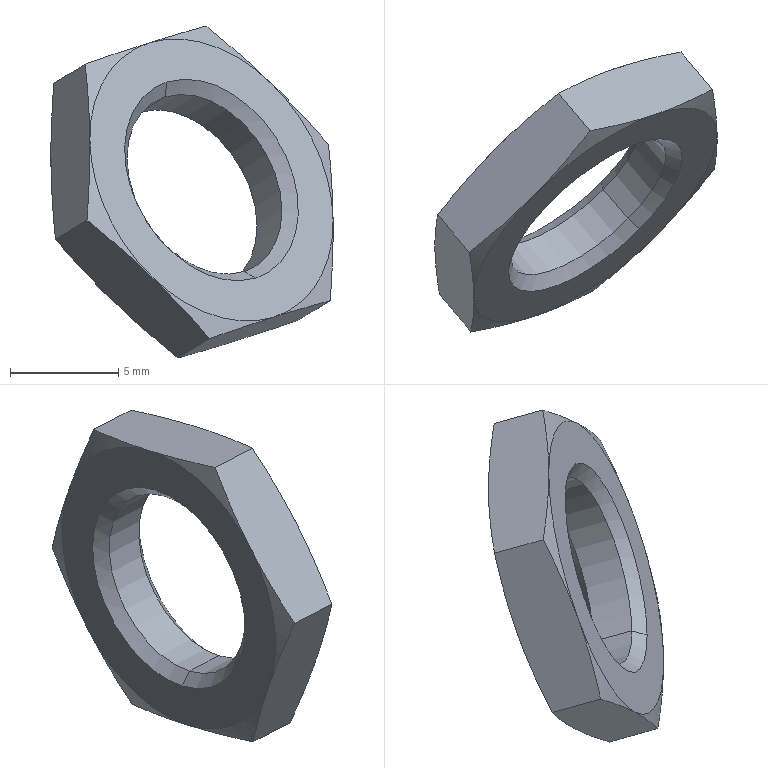Component | SolidWorks | SCPG-L-00-16-45-T0H-D-7_5-1 | 1 solid | 26 faces | box 13.01 x 12.91 x 15.3 mm | volume 310 mm3 | cone 16 | plane 8 | cylinder 2 | commonest cylinder face diameters 8.917 x2
STEP:
#1=COLOUR_RGB('',0.7922,0.8196,0.9333);
#2=FILL_AREA_STYLE_COLOUR('',#1);
#3=FILL_AREA_STYLE('',(#2));
#4=SURFACE_STYLE_FILL_AREA(#3);
#5=SURFACE_SIDE_STYLE('',(#4));
#6=SURFACE_STYLE_USAGE(.BOTH.,#5);
#7=PRESENTATION_STYLE_ASSIGNMENT((#6));
#8=CARTESIAN_POINT('',(17.404,-8.214,-2.973));
#9=VERTEX_POINT('',#8);
#10=CARTESIAN_POINT('',(17.548,-8.258,-3.29));
#11=VERTEX_POINT('',#10);
#12=CARTESIAN_POINT('',(17.476,-8.236,-3.132));
#13=DIRECTION('',(0.5985,-0.711,0.3692));
#14=DIRECTION('',(-0.6887,-0.692,-0.2163));
#15=AXIS2_PLACEMENT_3D('',#12,#13,#14);
#16=CIRCLE('',#15,0.1755);
#17=EDGE_CURVE('',#9,#11,#16,.T.);
#18=ORIENTED_EDGE('',*,*,#17,.F.);
#19=CARTESIAN_POINT('',(17.408,-8.226,-2.946));
#20=VERTEX_POINT('',#19);
#21=CARTESIAN_POINT('',(17.408,-8.226,-2.946));
#22=DIRECTION('',(0.1337,-0.4145,0.9002));
#23=VECTOR('',#22,39.37);
#24=LINE('',#21,#23);
#25=EDGE_CURVE('',#9,#20,#24,.T.);
#26=ORIENTED_EDGE('',*,*,#25,.T.);
#27=CARTESIAN_POINT('',(17.569,-8.275,-3.302));
#28=VERTEX_POINT('',#27);
#29=CARTESIAN_POINT('',(17.488,-8.251,-3.124));
#30=DIRECTION('',(-0.5985,0.711,-0.3692));
#31=DIRECTION('',(0.4093,-0.1248,-0.9038));
#32=AXIS2_PLACEMENT_3D('',#29,#30,#31);
#33=CIRCLE('',#32,0.1969);
#34=EDGE_CURVE('',#28,#20,#33,.T.);
#35=ORIENTED_EDGE('',*,*,#34,.F.);
#36=CARTESIAN_POINT('',(17.569,-8.275,-3.302));
#37=DIRECTION('',(0.7126,-0.591,-0.378));
#38=VECTOR('',#37,39.37);
#39=LINE('',#36,#38);
#40=EDGE_CURVE('',#11,#28,#39,.T.);
#41=ORIENTED_EDGE('',*,*,#40,.F.);
#42=EDGE_LOOP('',(#18,#26,#35,#41));
#43=FACE_OUTER_BOUND('',#42,.T.);
#44=CARTESIAN_POINT('',(17.488,-8.251,-3.124));
#45=DIRECTION('',(0.5985,-0.711,0.3692));
#46=DIRECTION('',(0.4093,-0.1248,-0.9038));
#47=AXIS2_PLACEMENT_3D('',#44,#45,#46);
#48=CONICAL_SURFACE('',#47,0.1969,0.7854);
#49=ADVANCED_FACE('',(#43),#48,.F.);
#50=ORIENTED_EDGE('',*,*,#17,.T.);
#51=CARTESIAN_POINT('',(17.502,-8.204,-3.318));
#52=VERTEX_POINT('',#51);
#53=CARTESIAN_POINT('',(17.525,-8.231,-3.304));
#54=DIRECTION('',(-0.5985,0.711,-0.3692));
#55=VECTOR('',#54,39.37);
#56=LINE('',#53,#55);
#57=EDGE_CURVE('',#11,#52,#56,.T.);
#58=ORIENTED_EDGE('',*,*,#57,.T.);
#59=CARTESIAN_POINT('',(17.359,-8.16,-3.001));
#60=VERTEX_POINT('',#59);
#61=CARTESIAN_POINT('',(17.43,-8.182,-3.159));
#62=DIRECTION('',(0.5985,-0.711,0.3692));
#63=DIRECTION('',(-0.4093,0.1248,0.9038));
#64=AXIS2_PLACEMENT_3D('',#61,#62,#63);
#65=CIRCLE('',#64,0.1755);
#66=EDGE_CURVE('',#60,#52,#65,.T.);
#67=ORIENTED_EDGE('',*,*,#66,.F.);
#68=CARTESIAN_POINT('',(17.381,-8.187,-2.987));
#69=DIRECTION('',(-0.5985,0.711,-0.3692));
#70=VECTOR('',#69,39.37);
#71=LINE('',#68,#70);
#72=EDGE_CURVE('',#9,#60,#71,.T.);
#73=ORIENTED_EDGE('',*,*,#72,.F.);
#74=EDGE_LOOP('',(#50,#58,#67,#73));
#75=FACE_OUTER_BOUND('',#74,.T.);
#76=CARTESIAN_POINT('',(17.453,-8.209,-3.146));
#77=DIRECTION('',(-0.5985,0.711,-0.3692));
#78=DIRECTION('',(-0.4093,0.1248,0.9038));
#79=AXIS2_PLACEMENT_3D('',#76,#77,#78);
#80=CYLINDRICAL_SURFACE('',#79,0.1755);
#81=ADVANCED_FACE('',(#75),#80,.F.);
#82=ORIENTED_EDGE('',*,*,#66,.T.);
#83=CARTESIAN_POINT('',(17.498,-8.191,-3.345));
#84=VERTEX_POINT('',#83);
#85=CARTESIAN_POINT('',(17.498,-8.191,-3.345));
#86=DIRECTION('',(-0.1337,0.4145,-0.9002));
#87=VECTOR('',#86,39.37);
#88=LINE('',#85,#87);
#89=EDGE_CURVE('',#52,#84,#88,.T.);
#90=ORIENTED_EDGE('',*,*,#89,.T.);
#91=CARTESIAN_POINT('',(17.337,-8.142,-2.989));
#92=VERTEX_POINT('',#91);
#93=CARTESIAN_POINT('',(17.418,-8.167,-3.167));
#94=DIRECTION('',(0.5985,-0.711,0.3692));
#95=DIRECTION('',(-0.4093,0.1248,0.9038));
#96=AXIS2_PLACEMENT_3D('',#93,#94,#95);
#97=CIRCLE('',#96,0.1969);
#98=EDGE_CURVE('',#92,#84,#97,.T.);
#99=ORIENTED_EDGE('',*,*,#98,.F.);
#100=CARTESIAN_POINT('',(17.337,-8.142,-2.989));
#101=DIRECTION('',(-0.7126,0.591,0.378));
#102=VECTOR('',#101,39.37);
#103=LINE('',#100,#102);
#104=EDGE_CURVE('',#60,#92,#103,.T.);
#105=ORIENTED_EDGE('',*,*,#104,.F.);
#106=EDGE_LOOP('',(#82,#90,#99,#105));
#107=FACE_OUTER_BOUND('',#106,.T.);
#108=CARTESIAN_POINT('',(17.418,-8.167,-3.167));
#109=DIRECTION('',(-0.5985,0.711,-0.3692));
#110=DIRECTION('',(-0.4093,0.1248,0.9038));
#111=AXIS2_PLACEMENT_3D('',#108,#109,#110);
#112=CONICAL_SURFACE('',#111,0.1969,0.7854);
#113=ADVANCED_FACE('',(#107),#112,.F.);
#114=CARTESIAN_POINT('',(17.596,-8.068,-2.948));
#115=VERTEX_POINT('',#114);
#116=CARTESIAN_POINT('',(17.376,-8.216,-2.875));
#117=VERTEX_POINT('',#116);
#118=CARTESIAN_POINT('',(17.488,-8.251,-3.124));
#119=DIRECTION('',(0.5985,-0.711,0.3692));
#120=DIRECTION('',(-0.4093,0.1248,0.9038));
#121=AXIS2_PLACEMENT_3D('',#118,#119,#120);
#122=CIRCLE('',#121,0.2756);
#123=EDGE_CURVE('',#115,#117,#122,.T.);
#124=ORIENTED_EDGE('',*,*,#123,.T.);
#125=CARTESIAN_POINT('',(17.268,-8.399,-3.051));
#126=VERTEX_POINT('',#125);
#127=CARTESIAN_POINT('',(17.488,-8.251,-3.124));
#128=DIRECTION('',(0.5985,-0.711,0.3692));
#129=DIRECTION('',(-0.4093,0.1248,0.9038));
#130=AXIS2_PLACEMENT_3D('',#127,#128,#129);
#131=CIRCLE('',#130,0.2756);
#132=EDGE_CURVE('',#117,#126,#131,.T.);
#133=ORIENTED_EDGE('',*,*,#132,.T.);
#134=CARTESIAN_POINT('',(17.38,-8.433,-3.3));
#135=VERTEX_POINT('',#134);
#136=CARTESIAN_POINT('',(17.488,-8.251,-3.124));
#137=DIRECTION('',(0.5985,-0.711,0.3692));
#138=DIRECTION('',(-0.4093,0.1248,0.9038));
#139=AXIS2_PLACEMENT_3D('',#136,#137,#138);
#140=CIRCLE('',#139,0.2756);
#141=EDGE_CURVE('',#126,#135,#140,.T.);
#142=ORIENTED_EDGE('',*,*,#141,.T.);
#143=CARTESIAN_POINT('',(17.601,-8.285,-3.373));
#144=VERTEX_POINT('',#143);
#145=CARTESIAN_POINT('',(17.488,-8.251,-3.124));
#146=DIRECTION('',(0.5985,-0.711,0.3692));
#147=DIRECTION('',(-0.4093,0.1248,0.9038));
#148=AXIS2_PLACEMENT_3D('',#145,#146,#147);
#149=CIRCLE('',#148,0.2756);
#150=EDGE_CURVE('',#135,#144,#149,.T.);
#151=ORIENTED_EDGE('',*,*,#150,.T.);
#152=CARTESIAN_POINT('',(17.709,-8.103,-3.197));
#153=VERTEX_POINT('',#152);
#154=CARTESIAN_POINT('',(17.488,-8.251,-3.124));
#155=DIRECTION('',(0.5985,-0.711,0.3692));
#156=DIRECTION('',(-0.4093,0.1248,0.9038));
#157=AXIS2_PLACEMENT_3D('',#154,#155,#156);
#158=CIRCLE('',#157,0.2756);
#159=EDGE_CURVE('',#144,#153,#158,.T.);
#160=ORIENTED_EDGE('',*,*,#159,.T.);
#161=CARTESIAN_POINT('',(17.488,-8.251,-3.124));
#162=DIRECTION('',(0.5985,-0.711,0.3692));
#163=DIRECTION('',(-0.4093,0.1248,0.9038));
#164=AXIS2_PLACEMENT_3D('',#161,#162,#163);
#165=CIRCLE('',#164,0.2756);
#166=EDGE_CURVE('',#153,#115,#165,.T.);
#167=ORIENTED_EDGE('',*,*,#166,.T.);
#168=EDGE_LOOP('',(#124,#133,#142,#151,#160,#167));
#169=FACE_OUTER_BOUND('',#168,.T.);
#170=ORIENTED_EDGE('',*,*,#34,.T.);
#171=CARTESIAN_POINT('',(17.488,-8.251,-3.124));
#172=DIRECTION('',(-0.5985,0.711,-0.3692));
#173=DIRECTION('',(0.4093,-0.1248,-0.9038));
#174=AXIS2_PLACEMENT_3D('',#171,#172,#173);
#175=CIRCLE('',#174,0.1969);
#176=EDGE_CURVE('',#20,#28,#175,.T.);
#177=ORIENTED_EDGE('',*,*,#176,.T.);
#178=EDGE_LOOP('',(#170,#177));
#179=FACE_BOUND('',#178,.T.);
#180=CARTESIAN_POINT('',(17.394,-8.346,-3.154));
#181=DIRECTION('',(0.5985,-0.711,0.3692));
#182=DIRECTION('',(0.4093,-0.1248,-0.9038));
#183=AXIS2_PLACEMENT_3D('',#180,#181,#182);
#184=PLANE('',#183);
#185=ADVANCED_FACE('',(#169,#179),#184,.T.);
#186=CARTESIAN_POINT('',(17.259,-8.318,-2.913));
#187=VERTEX_POINT('',#186);
#188=CARTESIAN_POINT('',(17.259,-8.318,-2.913));
#189=CARTESIAN_POINT('',(17.264,-8.347,-2.958));
#190=CARTESIAN_POINT('',(17.267,-8.375,-3.003));
#191=CARTESIAN_POINT('',(17.268,-8.399,-3.051));
#192=B_SPLINE_CURVE_WITH_KNOTS('',3,(#188,#189,#190,#191),.UNSPECIFIED.,.F.,.F.,(4,4),(0.,0.004052),.UNSPECIFIED.);
#193=EDGE_CURVE('',#187,#126,#192,.T.);
#194=ORIENTED_EDGE('',*,*,#193,.T.);
#195=ORIENTED_EDGE('',*,*,#132,.F.);
#196=CARTESIAN_POINT('',(17.376,-8.216,-2.875));
#197=CARTESIAN_POINT('',(17.339,-8.253,-2.886));
#198=CARTESIAN_POINT('',(17.3,-8.287,-2.899));
#199=CARTESIAN_POINT('',(17.259,-8.318,-2.913));
#200=B_SPLINE_CURVE_WITH_KNOTS('',3,(#196,#197,#198,#199),.UNSPECIFIED.,.F.,.F.,(4,4),(0.,0.004052),.UNSPECIFIED.);
#201=EDGE_CURVE('',#117,#187,#200,.T.);
#202=ORIENTED_EDGE('',*,*,#201,.T.);
#203=EDGE_LOOP('',(#194,#195,#202));
#204=FACE_OUTER_BOUND('',#203,.T.);
#205=CARTESIAN_POINT('',(17.482,-8.243,-3.128));
#206=DIRECTION('',(-0.5985,0.711,-0.3692));
#207=DIRECTION('',(-0.4093,0.1248,0.9038));
#208=AXIS2_PLACEMENT_3D('',#205,#206,#207);
#209=CONICAL_SURFACE('',#208,0.3185,1.309);
#210=ADVANCED_FACE('',(#204),#209,.T.);
#211=CARTESIAN_POINT('',(17.478,-8.098,-2.844));
#212=VERTEX_POINT('',#211);
#213=CARTESIAN_POINT('',(17.478,-8.098,-2.844));
#214=CARTESIAN_POINT('',(17.446,-8.14,-2.853));
#215=CARTESIAN_POINT('',(17.412,-8.179,-2.863));
#216=CARTESIAN_POINT('',(17.376,-8.216,-2.875));
#217=B_SPLINE_CURVE_WITH_KNOTS('',3,(#213,#214,#215,#216),.UNSPECIFIED.,.F.,.F.,(4,4),(0.,0.004052),.UNSPECIFIED.);
#218=EDGE_CURVE('',#212,#117,#217,.T.);
#219=ORIENTED_EDGE('',*,*,#218,.T.);
#220=ORIENTED_EDGE('',*,*,#123,.F.);
#221=CARTESIAN_POINT('',(17.596,-8.068,-2.948));
#222=CARTESIAN_POINT('',(17.559,-8.081,-2.912));
#223=CARTESIAN_POINT('',(17.519,-8.091,-2.877));
#224=CARTESIAN_POINT('',(17.478,-8.098,-2.844));
#225=B_SPLINE_CURVE_WITH_KNOTS('',3,(#221,#222,#223,#224),.UNSPECIFIED.,.F.,.F.,(4,4),(0.,0.004052),.UNSPECIFIED.);
#226=EDGE_CURVE('',#115,#212,#225,.T.);
#227=ORIENTED_EDGE('',*,*,#226,.T.);
#228=EDGE_LOOP('',(#219,#220,#227));
#229=FACE_OUTER_BOUND('',#228,.T.);
#230=CARTESIAN_POINT('',(17.482,-8.243,-3.128));
#231=DIRECTION('',(-0.5985,0.711,-0.3692));
#232=DIRECTION('',(-0.4093,0.1248,0.9038));
#233=AXIS2_PLACEMENT_3D('',#230,#231,#232);
#234=CONICAL_SURFACE('',#233,0.3185,1.309);
#235=ADVANCED_FACE('',(#229),#234,.T.);
#236=CARTESIAN_POINT('',(17.701,-8.022,-3.059));
#237=VERTEX_POINT('',#236);
#238=CARTESIAN_POINT('',(17.701,-8.022,-3.059));
#239=CARTESIAN_POINT('',(17.668,-8.04,-3.021));
#240=CARTESIAN_POINT('',(17.634,-8.056,-2.983));
#241=CARTESIAN_POINT('',(17.596,-8.068,-2.948));
#242=B_SPLINE_CURVE_WITH_KNOTS('',3,(#238,#239,#240,#241),.UNSPECIFIED.,.F.,.F.,(4,4),(0.,0.004052),.UNSPECIFIED.);
#243=EDGE_CURVE('',#237,#115,#242,.T.);
#244=ORIENTED_EDGE('',*,*,#243,.T.);
#245=ORIENTED_EDGE('',*,*,#166,.F.);
#246=CARTESIAN_POINT('',(17.709,-8.103,-3.197));
#247=CARTESIAN_POINT('',(17.709,-8.079,-3.149));
#248=CARTESIAN_POINT('',(17.706,-8.051,-3.104));
#249=CARTESIAN_POINT('',(17.701,-8.022,-3.059));
#250=B_SPLINE_CURVE_WITH_KNOTS('',3,(#246,#247,#248,#249),.UNSPECIFIED.,.F.,.F.,(4,4),(0.,0.004052),.UNSPECIFIED.);
#251=EDGE_CURVE('',#153,#237,#250,.T.);
#252=ORIENTED_EDGE('',*,*,#251,.T.);
#253=EDGE_LOOP('',(#244,#245,#252));
#254=FACE_OUTER_BOUND('',#253,.T.);
#255=CARTESIAN_POINT('',(17.482,-8.243,-3.128));
#256=DIRECTION('',(-0.5985,0.711,-0.3692));
#257=DIRECTION('',(-0.4093,0.1248,0.9038));
#258=AXIS2_PLACEMENT_3D('',#255,#256,#257);
#259=CONICAL_SURFACE('',#258,0.3185,1.309);
#260=ADVANCED_FACE('',(#254),#259,.T.);
#261=ORIENTED_EDGE('',*,*,#159,.F.);
#262=CARTESIAN_POINT('',(17.704,-8.167,-3.343));
#263=VERTEX_POINT('',#262);
#264=CARTESIAN_POINT('',(17.601,-8.285,-3.373));
#265=CARTESIAN_POINT('',(17.638,-8.248,-3.361));
#266=CARTESIAN_POINT('',(17.672,-8.209,-3.351));
#267=CARTESIAN_POINT('',(17.704,-8.167,-3.343));
#268=B_SPLINE_CURVE_WITH_KNOTS('',3,(#264,#265,#266,#267),.UNSPECIFIED.,.F.,.F.,(4,4),(0.,0.004052),.UNSPECIFIED.);
#269=EDGE_CURVE('',#144,#263,#268,.T.);
#270=ORIENTED_EDGE('',*,*,#269,.T.);
#271=CARTESIAN_POINT('',(17.704,-8.167,-3.343));
#272=CARTESIAN_POINT('',(17.708,-8.148,-3.293));
#273=CARTESIAN_POINT('',(17.71,-8.127,-3.244));
#274=CARTESIAN_POINT('',(17.709,-8.103,-3.197));
#275=B_SPLINE_CURVE_WITH_KNOTS('',3,(#271,#272,#273,#274),.UNSPECIFIED.,.F.,.F.,(4,4),(0.,0.004052),.UNSPECIFIED.);
#276=EDGE_CURVE('',#263,#153,#275,.T.);
#277=ORIENTED_EDGE('',*,*,#276,.T.);
#278=EDGE_LOOP('',(#261,#270,#277));
#279=FACE_OUTER_BOUND('',#278,.T.);
#280=CARTESIAN_POINT('',(17.482,-8.243,-3.128));
#281=DIRECTION('',(-0.5985,0.711,-0.3692));
#282=DIRECTION('',(-0.4093,0.1248,0.9038));
#283=AXIS2_PLACEMENT_3D('',#280,#281,#282);
#284=CONICAL_SURFACE('',#283,0.3185,1.309);
#285=ADVANCED_FACE('',(#279),#284,.T.);
#286=ORIENTED_EDGE('',*,*,#150,.F.);
#287=CARTESIAN_POINT('',(17.485,-8.387,-3.411));
#288=VERTEX_POINT('',#287);
#289=CARTESIAN_POINT('',(17.38,-8.433,-3.3));
#290=CARTESIAN_POINT('',(17.418,-8.42,-3.336));
#291=CARTESIAN_POINT('',(17.452,-8.405,-3.373));
#292=CARTESIAN_POINT('',(17.485,-8.387,-3.411));
#293=B_SPLINE_CURVE_WITH_KNOTS('',3,(#289,#290,#291,#292),.UNSPECIFIED.,.F.,.F.,(4,4),(0.,0.004052),.UNSPECIFIED.);
#294=EDGE_CURVE('',#135,#288,#293,.T.);
#295=ORIENTED_EDGE('',*,*,#294,.T.);
#296=CARTESIAN_POINT('',(17.485,-8.387,-3.411));
#297=CARTESIAN_POINT('',(17.525,-8.356,-3.397));
#298=CARTESIAN_POINT('',(17.565,-8.322,-3.384));
#299=CARTESIAN_POINT('',(17.601,-8.285,-3.373));
#300=B_SPLINE_CURVE_WITH_KNOTS('',3,(#296,#297,#298,#299),.UNSPECIFIED.,.F.,.F.,(4,4),(0.,0.004052),.UNSPECIFIED.);
#301=EDGE_CURVE('',#288,#144,#300,.T.);
#302=ORIENTED_EDGE('',*,*,#301,.T.);
#303=EDGE_LOOP('',(#286,#295,#302));
#304=FACE_OUTER_BOUND('',#303,.T.);
#305=CARTESIAN_POINT('',(17.482,-8.243,-3.128));
#306=DIRECTION('',(-0.5985,0.711,-0.3692));
#307=DIRECTION('',(-0.4093,0.1248,0.9038));
#308=AXIS2_PLACEMENT_3D('',#305,#306,#307);
#309=CONICAL_SURFACE('',#308,0.3185,1.309);
#310=ADVANCED_FACE('',(#304),#309,.T.);
#311=CARTESIAN_POINT('',(17.262,-8.463,-3.197));
#312=VERTEX_POINT('',#311);
#313=CARTESIAN_POINT('',(17.262,-8.463,-3.197));
#314=CARTESIAN_POINT('',(17.304,-8.455,-3.23));
#315=CARTESIAN_POINT('',(17.343,-8.446,-3.264));
#316=CARTESIAN_POINT('',(17.38,-8.433,-3.3));
#317=B_SPLINE_CURVE_WITH_KNOTS('',3,(#313,#314,#315,#316),.UNSPECIFIED.,.F.,.F.,(4,4),(0.,0.004052),.UNSPECIFIED.);
#318=EDGE_CURVE('',#312,#135,#317,.T.);
#319=ORIENTED_EDGE('',*,*,#318,.T.);
#320=ORIENTED_EDGE('',*,*,#141,.F.);
#321=CARTESIAN_POINT('',(17.268,-8.399,-3.051));
#322=CARTESIAN_POINT('',(17.268,-8.423,-3.098));
#323=CARTESIAN_POINT('',(17.266,-8.444,-3.147));
#324=CARTESIAN_POINT('',(17.262,-8.463,-3.197));
#325=B_SPLINE_CURVE_WITH_KNOTS('',3,(#321,#322,#323,#324),.UNSPECIFIED.,.F.,.F.,(4,4),(0.,0.004052),.UNSPECIFIED.);
#326=EDGE_CURVE('',#126,#312,#325,.T.);
#327=ORIENTED_EDGE('',*,*,#326,.T.);
#328=EDGE_LOOP('',(#319,#320,#327));
#329=FACE_OUTER_BOUND('',#328,.T.);
#330=CARTESIAN_POINT('',(17.482,-8.243,-3.128));
#331=DIRECTION('',(-0.5985,0.711,-0.3692));
#332=DIRECTION('',(-0.4093,0.1248,0.9038));
#333=AXIS2_PLACEMENT_3D('',#330,#331,#332);
#334=CONICAL_SURFACE('',#333,0.3185,1.309);
#335=ADVANCED_FACE('',(#329),#334,.T.);
#336=ORIENTED_EDGE('',*,*,#25,.F.);
#337=CARTESIAN_POINT('',(17.476,-8.236,-3.132));
#338=DIRECTION('',(0.5985,-0.711,0.3692));
#339=DIRECTION('',(-0.6887,-0.692,-0.2163));
#340=AXIS2_PLACEMENT_3D('',#337,#338,#339);
#341=CIRCLE('',#340,0.1755);
#342=EDGE_CURVE('',#11,#9,#341,.T.);
#343=ORIENTED_EDGE('',*,*,#342,.F.);
#344=ORIENTED_EDGE('',*,*,#40,.T.);
#345=ORIENTED_EDGE('',*,*,#176,.F.);
#346=EDGE_LOOP('',(#336,#343,#344,#345));
#347=FACE_OUTER_BOUND('',#346,.T.);
#348=CARTESIAN_POINT('',(17.488,-8.251,-3.124));
#349=DIRECTION('',(0.5985,-0.711,0.3692));
#350=DIRECTION('',(0.4093,-0.1248,-0.9038));
#351=AXIS2_PLACEMENT_3D('',#348,#349,#350);
#352=CONICAL_SURFACE('',#351,0.1969,0.7854);
#353=ADVANCED_FACE('',(#347),#352,.F.);
#354=CARTESIAN_POINT('',(17.205,-8.395,-3.232));
#355=VERTEX_POINT('',#354);
#356=CARTESIAN_POINT('',(17.269,-8.471,-3.193));
#357=DIRECTION('',(-0.5985,0.711,-0.3692));
#358=VECTOR('',#357,39.37);
#359=LINE('',#356,#358);
#360=EDGE_CURVE('',#312,#355,#359,.T.);
#361=ORIENTED_EDGE('',*,*,#360,.F.);
#362=ORIENTED_EDGE('',*,*,#326,.F.);
#363=ORIENTED_EDGE('',*,*,#193,.F.);
#364=CARTESIAN_POINT('',(17.202,-8.251,-2.948));
#365=VERTEX_POINT('',#364);
#366=CARTESIAN_POINT('',(17.266,-8.326,-2.909));
#367=DIRECTION('',(0.5985,-0.711,0.3692));
#368=VECTOR('',#367,39.37);
#369=LINE('',#366,#368);
#370=EDGE_CURVE('',#365,#187,#369,.T.);
#371=ORIENTED_EDGE('',*,*,#370,.F.);
#372=CARTESIAN_POINT('',(17.197,-8.315,-3.094));
#373=VERTEX_POINT('',#372);
#374=CARTESIAN_POINT('',(17.197,-8.315,-3.094));
#375=CARTESIAN_POINT('',(17.196,-8.291,-3.047));
#376=CARTESIAN_POINT('',(17.198,-8.27,-2.998));
#377=CARTESIAN_POINT('',(17.202,-8.251,-2.948));
#378=B_SPLINE_CURVE_WITH_KNOTS('',3,(#374,#375,#376,#377),.UNSPECIFIED.,.F.,.F.,(4,4),(0.,0.004052),.UNSPECIFIED.);
#379=EDGE_CURVE('',#373,#365,#378,.T.);
#380=ORIENTED_EDGE('',*,*,#379,.F.);
#381=CARTESIAN_POINT('',(17.205,-8.395,-3.232));
#382=CARTESIAN_POINT('',(17.201,-8.366,-3.188));
#383=CARTESIAN_POINT('',(17.198,-8.339,-3.142));
#384=CARTESIAN_POINT('',(17.197,-8.315,-3.094));
#385=B_SPLINE_CURVE_WITH_KNOTS('',3,(#381,#382,#383,#384),.UNSPECIFIED.,.F.,.F.,(4,4),(0.,0.004052),.UNSPECIFIED.);
#386=EDGE_CURVE('',#355,#373,#385,.T.);
#387=ORIENTED_EDGE('',*,*,#386,.F.);
#388=EDGE_LOOP('',(#361,#362,#363,#371,#380,#387));
#389=FACE_OUTER_BOUND('',#388,.T.);
#390=CARTESIAN_POINT('',(17.269,-8.471,-3.193));
#391=DIRECTION('',(0.8011,0.5369,-0.2645));
#392=DIRECTION('',(0.01014,-0.4541,-0.8909));
#393=AXIS2_PLACEMENT_3D('',#390,#391,#392);
#394=PLANE('',#393);
#395=ADVANCED_FACE('',(#389),#394,.F.);
#396=CARTESIAN_POINT('',(17.305,-8.132,-2.918));
#397=VERTEX_POINT('',#396);
#398=CARTESIAN_POINT('',(17.202,-8.251,-2.948));
#399=CARTESIAN_POINT('',(17.234,-8.209,-2.94));
#400=CARTESIAN_POINT('',(17.268,-8.169,-2.93));
#401=CARTESIAN_POINT('',(17.305,-8.132,-2.918));
#402=B_SPLINE_CURVE_WITH_KNOTS('',3,(#398,#399,#400,#401),.UNSPECIFIED.,.F.,.F.,(4,4),(0.,0.004052),.UNSPECIFIED.);
#403=EDGE_CURVE('',#365,#397,#402,.T.);
#404=ORIENTED_EDGE('',*,*,#403,.F.);
#405=ORIENTED_EDGE('',*,*,#370,.T.);
#406=ORIENTED_EDGE('',*,*,#201,.F.);
#407=ORIENTED_EDGE('',*,*,#218,.F.);
#408=CARTESIAN_POINT('',(17.421,-8.03,-2.88));
#409=VERTEX_POINT('',#408);
#410=CARTESIAN_POINT('',(17.485,-8.106,-2.84));
#411=DIRECTION('',(0.5985,-0.711,0.3692));
#412=VECTOR('',#411,39.37);
#413=LINE('',#410,#412);
#414=EDGE_CURVE('',#409,#212,#413,.T.);
#415=ORIENTED_EDGE('',*,*,#414,.F.);
#416=CARTESIAN_POINT('',(17.305,-8.132,-2.918));
#417=CARTESIAN_POINT('',(17.342,-8.096,-2.907));
#418=CARTESIAN_POINT('',(17.381,-8.062,-2.894));
#419=CARTESIAN_POINT('',(17.421,-8.03,-2.88));
#420=B_SPLINE_CURVE_WITH_KNOTS('',3,(#416,#417,#418,#419),.UNSPECIFIED.,.F.,.F.,(4,4),(0.,0.004052),.UNSPECIFIED.);
#421=EDGE_CURVE('',#397,#409,#420,.T.);
#422=ORIENTED_EDGE('',*,*,#421,.F.);
#423=EDGE_LOOP('',(#404,#405,#406,#407,#415,#422));
#424=FACE_OUTER_BOUND('',#423,.T.);
#425=CARTESIAN_POINT('',(17.266,-8.326,-2.909));
#426=DIRECTION('',(0.4093,-0.1248,-0.9038));
#427=DIRECTION('',(-0.5985,0.711,-0.3692));
#428=AXIS2_PLACEMENT_3D('',#425,#426,#427);
#429=PLANE('',#428);
#430=ADVANCED_FACE('',(#424),#429,.F.);
#431=CARTESIAN_POINT('',(17.526,-7.984,-2.991));
#432=VERTEX_POINT('',#431);
#433=CARTESIAN_POINT('',(17.421,-8.03,-2.88));
#434=CARTESIAN_POINT('',(17.454,-8.013,-2.918));
#435=CARTESIAN_POINT('',(17.488,-7.997,-2.955));
#436=CARTESIAN_POINT('',(17.526,-7.984,-2.991));
#437=B_SPLINE_CURVE_WITH_KNOTS('',3,(#433,#434,#435,#436),.UNSPECIFIED.,.F.,.F.,(4,4),(0.,0.004052),.UNSPECIFIED.);
#438=EDGE_CURVE('',#409,#432,#437,.T.);
#439=ORIENTED_EDGE('',*,*,#438,.F.);
#440=ORIENTED_EDGE('',*,*,#414,.T.);
#441=ORIENTED_EDGE('',*,*,#226,.F.);
#442=ORIENTED_EDGE('',*,*,#243,.F.);
#443=CARTESIAN_POINT('',(17.644,-7.955,-3.094));
#444=VERTEX_POINT('',#443);
#445=CARTESIAN_POINT('',(17.708,-8.031,-3.055));
#446=DIRECTION('',(0.5985,-0.711,0.3692));
#447=VECTOR('',#446,39.37);
#448=LINE('',#445,#447);
#449=EDGE_CURVE('',#444,#237,#448,.T.);
#450=ORIENTED_EDGE('',*,*,#449,.F.);
#451=CARTESIAN_POINT('',(17.526,-7.984,-2.991));
#452=CARTESIAN_POINT('',(17.563,-7.972,-3.027));
#453=CARTESIAN_POINT('',(17.603,-7.962,-3.061));
#454=CARTESIAN_POINT('',(17.644,-7.955,-3.094));
#455=B_SPLINE_CURVE_WITH_KNOTS('',3,(#451,#452,#453,#454),.UNSPECIFIED.,.F.,.F.,(4,4),(0.,0.004052),.UNSPECIFIED.);
#456=EDGE_CURVE('',#432,#444,#455,.T.);
#457=ORIENTED_EDGE('',*,*,#456,.F.);
#458=EDGE_LOOP('',(#439,#440,#441,#442,#450,#457));
#459=FACE_OUTER_BOUND('',#458,.T.);
#460=CARTESIAN_POINT('',(17.485,-8.106,-2.84));
#461=DIRECTION('',(-0.3918,-0.6617,-0.6393));
#462=DIRECTION('',(-0.6988,-0.2379,0.6745));
#463=AXIS2_PLACEMENT_3D('',#460,#461,#462);
#464=PLANE('',#463);
#465=ADVANCED_FACE('',(#459),#464,.F.);
#466=CARTESIAN_POINT('',(17.639,-8.019,-3.24));
#467=VERTEX_POINT('',#466);
#468=CARTESIAN_POINT('',(17.644,-7.955,-3.094));
#469=CARTESIAN_POINT('',(17.64,-7.974,-3.144));
#470=CARTESIAN_POINT('',(17.638,-7.995,-3.193));
#471=CARTESIAN_POINT('',(17.639,-8.019,-3.24));
#472=B_SPLINE_CURVE_WITH_KNOTS('',3,(#468,#469,#470,#471),.UNSPECIFIED.,.F.,.F.,(4,4),(0.,0.004052),.UNSPECIFIED.);
#473=EDGE_CURVE('',#444,#467,#472,.T.);
#474=ORIENTED_EDGE('',*,*,#473,.F.);
#475=ORIENTED_EDGE('',*,*,#449,.T.);
#476=ORIENTED_EDGE('',*,*,#251,.F.);
#477=ORIENTED_EDGE('',*,*,#276,.F.);
#478=CARTESIAN_POINT('',(17.647,-8.099,-3.378));
#479=VERTEX_POINT('',#478);
#480=CARTESIAN_POINT('',(17.711,-8.175,-3.338));
#481=DIRECTION('',(0.5985,-0.711,0.3692));
#482=VECTOR('',#481,39.37);
#483=LINE('',#480,#482);
#484=EDGE_CURVE('',#479,#263,#483,.T.);
#485=ORIENTED_EDGE('',*,*,#484,.F.);
#486=CARTESIAN_POINT('',(17.639,-8.019,-3.24));
#487=CARTESIAN_POINT('',(17.639,-8.043,-3.288));
#488=CARTESIAN_POINT('',(17.642,-8.07,-3.333));
#489=CARTESIAN_POINT('',(17.647,-8.099,-3.378));
#490=B_SPLINE_CURVE_WITH_KNOTS('',3,(#486,#487,#488,#489),.UNSPECIFIED.,.F.,.F.,(4,4),(0.,0.004052),.UNSPECIFIED.);
#491=EDGE_CURVE('',#467,#479,#490,.T.);
#492=ORIENTED_EDGE('',*,*,#491,.F.);
#493=EDGE_LOOP('',(#474,#475,#476,#477,#485,#492));
#494=FACE_OUTER_BOUND('',#493,.T.);
#495=CARTESIAN_POINT('',(17.708,-8.031,-3.055));
#496=DIRECTION('',(-0.8011,-0.5369,0.2645));
#497=DIRECTION('',(-0.01014,0.4541,0.8909));
#498=AXIS2_PLACEMENT_3D('',#495,#496,#497);
#499=PLANE('',#498);
#500=ADVANCED_FACE('',(#494),#499,.F.);
#501=ORIENTED_EDGE('',*,*,#484,.T.);
#502=ORIENTED_EDGE('',*,*,#269,.F.);
#503=ORIENTED_EDGE('',*,*,#301,.F.);
#504=CARTESIAN_POINT('',(17.428,-8.319,-3.447));
#505=VERTEX_POINT('',#504);
#506=CARTESIAN_POINT('',(17.492,-8.395,-3.407));
#507=DIRECTION('',(0.5985,-0.711,0.3692));
#508=VECTOR('',#507,39.37);
#509=LINE('',#506,#508);
#510=EDGE_CURVE('',#505,#288,#509,.T.);
#511=ORIENTED_EDGE('',*,*,#510,.F.);
#512=CARTESIAN_POINT('',(17.531,-8.201,-3.416));
#513=VERTEX_POINT('',#512);
#514=CARTESIAN_POINT('',(17.531,-8.201,-3.416));
#515=CARTESIAN_POINT('',(17.494,-8.238,-3.428));
#516=CARTESIAN_POINT('',(17.46,-8.278,-3.438));
#517=CARTESIAN_POINT('',(17.428,-8.319,-3.447));
#518=B_SPLINE_CURVE_WITH_KNOTS('',3,(#514,#515,#516,#517),.UNSPECIFIED.,.F.,.F.,(4,4),(0.,0.004052),.UNSPECIFIED.);
#519=EDGE_CURVE('',#513,#505,#518,.T.);
#520=ORIENTED_EDGE('',*,*,#519,.F.);
#521=CARTESIAN_POINT('',(17.647,-8.099,-3.378));
#522=CARTESIAN_POINT('',(17.606,-8.131,-3.392));
#523=CARTESIAN_POINT('',(17.567,-8.164,-3.405));
#524=CARTESIAN_POINT('',(17.531,-8.201,-3.416));
#525=B_SPLINE_CURVE_WITH_KNOTS('',3,(#521,#522,#523,#524),.UNSPECIFIED.,.F.,.F.,(4,4),(0.,0.004052),.UNSPECIFIED.);
#526=EDGE_CURVE('',#479,#513,#525,.T.);
#527=ORIENTED_EDGE('',*,*,#526,.F.);
#528=EDGE_LOOP('',(#501,#502,#503,#511,#520,#527));
#529=FACE_OUTER_BOUND('',#528,.T.);
#530=CARTESIAN_POINT('',(17.711,-8.175,-3.338));
#531=DIRECTION('',(-0.4093,0.1248,0.9038));
#532=DIRECTION('',(0.5985,-0.711,0.3692));
#533=AXIS2_PLACEMENT_3D('',#530,#531,#532);
#534=PLANE('',#533);
#535=ADVANCED_FACE('',(#529),#534,.F.);
#536=ORIENTED_EDGE('',*,*,#510,.T.);
#537=ORIENTED_EDGE('',*,*,#294,.F.);
#538=ORIENTED_EDGE('',*,*,#318,.F.);
#539=ORIENTED_EDGE('',*,*,#360,.T.);
#540=CARTESIAN_POINT('',(17.31,-8.349,-3.343));
#541=VERTEX_POINT('',#540);
#542=CARTESIAN_POINT('',(17.31,-8.349,-3.343));
#543=CARTESIAN_POINT('',(17.273,-8.362,-3.308));
#544=CARTESIAN_POINT('',(17.238,-8.378,-3.27));
#545=CARTESIAN_POINT('',(17.205,-8.395,-3.232));
#546=B_SPLINE_CURVE_WITH_KNOTS('',3,(#542,#543,#544,#545),.UNSPECIFIED.,.F.,.F.,(4,4),(0.,0.004052),.UNSPECIFIED.);
#547=EDGE_CURVE('',#541,#355,#546,.T.);
#548=ORIENTED_EDGE('',*,*,#547,.F.);
#549=CARTESIAN_POINT('',(17.428,-8.319,-3.447));
#550=CARTESIAN_POINT('',(17.387,-8.327,-3.414));
#551=CARTESIAN_POINT('',(17.347,-8.336,-3.379));
#552=CARTESIAN_POINT('',(17.31,-8.349,-3.343));
#553=B_SPLINE_CURVE_WITH_KNOTS('',3,(#549,#550,#551,#552),.UNSPECIFIED.,.F.,.F.,(4,4),(0.,0.004052),.UNSPECIFIED.);
#554=EDGE_CURVE('',#505,#541,#553,.T.);
#555=ORIENTED_EDGE('',*,*,#554,.F.);
#556=EDGE_LOOP('',(#536,#537,#538,#539,#548,#555));
#557=FACE_OUTER_BOUND('',#556,.T.);
#558=CARTESIAN_POINT('',(17.492,-8.395,-3.407));
#559=DIRECTION('',(0.3918,0.6617,0.6393));
#560=DIRECTION('',(0.6988,0.2379,-0.6745));
#561=AXIS2_PLACEMENT_3D('',#558,#559,#560);
#562=PLANE('',#561);
#563=ADVANCED_FACE('',(#557),#562,.F.);
#564=ORIENTED_EDGE('',*,*,#57,.F.);
#565=ORIENTED_EDGE('',*,*,#342,.T.);
#566=ORIENTED_EDGE('',*,*,#72,.T.);
#567=CARTESIAN_POINT('',(17.43,-8.182,-3.159));
#568=DIRECTION('',(0.5985,-0.711,0.3692));
#569=DIRECTION('',(-0.4093,0.1248,0.9038));
#570=AXIS2_PLACEMENT_3D('',#567,#568,#569);
#571=CIRCLE('',#570,0.1755);
#572=EDGE_CURVE('',#52,#60,#571,.T.);
#573=ORIENTED_EDGE('',*,*,#572,.F.);
#574=EDGE_LOOP('',(#564,#565,#566,#573));
#575=FACE_OUTER_BOUND('',#574,.T.);
#576=CARTESIAN_POINT('',(17.453,-8.209,-3.146));
#577=DIRECTION('',(-0.5985,0.711,-0.3692));
#578=DIRECTION('',(-0.4093,0.1248,0.9038));
#579=AXIS2_PLACEMENT_3D('',#576,#577,#578);
#580=CYLINDRICAL_SURFACE('',#579,0.1755);
#581=ADVANCED_FACE('',(#575),#580,.F.);
#582=ORIENTED_EDGE('',*,*,#386,.T.);
#583=CARTESIAN_POINT('',(17.418,-8.167,-3.167));
#584=DIRECTION('',(0.5985,-0.711,0.3692));
#585=DIRECTION('',(0.4093,-0.1248,-0.9038));
#586=AXIS2_PLACEMENT_3D('',#583,#584,#585);
#587=CIRCLE('',#586,0.2756);
#588=EDGE_CURVE('',#373,#541,#587,.T.);
#589=ORIENTED_EDGE('',*,*,#588,.T.);
#590=ORIENTED_EDGE('',*,*,#547,.T.);
#591=EDGE_LOOP('',(#582,#589,#590));
#592=FACE_OUTER_BOUND('',#591,.T.);
#593=CARTESIAN_POINT('',(17.425,-8.175,-3.163));
#594=DIRECTION('',(0.5985,-0.711,0.3692));
#595=DIRECTION('',(0.4093,-0.1248,-0.9038));
#596=AXIS2_PLACEMENT_3D('',#593,#594,#595);
#597=CONICAL_SURFACE('',#596,0.3185,1.309);
#598=ADVANCED_FACE('',(#592),#597,.T.);
#599=ORIENTED_EDGE('',*,*,#403,.T.);
#600=CARTESIAN_POINT('',(17.418,-8.167,-3.167));
#601=DIRECTION('',(0.5985,-0.711,0.3692));
#602=DIRECTION('',(0.4093,-0.1248,-0.9038));
#603=AXIS2_PLACEMENT_3D('',#600,#601,#602);
#604=CIRCLE('',#603,0.2756);
#605=EDGE_CURVE('',#397,#373,#604,.T.);
#606=ORIENTED_EDGE('',*,*,#605,.T.);
#607=ORIENTED_EDGE('',*,*,#379,.T.);
#608=EDGE_LOOP('',(#599,#606,#607));
#609=FACE_OUTER_BOUND('',#608,.T.);
#610=CARTESIAN_POINT('',(17.425,-8.175,-3.163));
#611=DIRECTION('',(0.5985,-0.711,0.3692));
#612=DIRECTION('',(0.4093,-0.1248,-0.9038));
#613=AXIS2_PLACEMENT_3D('',#610,#611,#612);
#614=CONICAL_SURFACE('',#613,0.3185,1.309);
#615=ADVANCED_FACE('',(#609),#614,.T.);
#616=CARTESIAN_POINT('',(17.418,-8.167,-3.167));
#617=DIRECTION('',(0.5985,-0.711,0.3692));
#618=DIRECTION('',(0.4093,-0.1248,-0.9038));
#619=AXIS2_PLACEMENT_3D('',#616,#617,#618);
#620=CIRCLE('',#619,0.2756);
#621=EDGE_CURVE('',#432,#397,#620,.T.);
#622=ORIENTED_EDGE('',*,*,#621,.T.);
#623=ORIENTED_EDGE('',*,*,#421,.T.);
#624=ORIENTED_EDGE('',*,*,#438,.T.);
#625=EDGE_LOOP('',(#622,#623,#624));
#626=FACE_OUTER_BOUND('',#625,.T.);
#627=CARTESIAN_POINT('',(17.425,-8.175,-3.163));
#628=DIRECTION('',(0.5985,-0.711,0.3692));
#629=DIRECTION('',(0.4093,-0.1248,-0.9038));
#630=AXIS2_PLACEMENT_3D('',#627,#628,#629);
#631=CONICAL_SURFACE('',#630,0.3185,1.309);
#632=ADVANCED_FACE('',(#626),#631,.T.);
#633=CARTESIAN_POINT('',(17.418,-8.167,-3.167));
#634=DIRECTION('',(0.5985,-0.711,0.3692));
#635=DIRECTION('',(0.4093,-0.1248,-0.9038));
#636=AXIS2_PLACEMENT_3D('',#633,#634,#635);
#637=CIRCLE('',#636,0.2756);
#638=EDGE_CURVE('',#467,#432,#637,.T.);
#639=ORIENTED_EDGE('',*,*,#638,.T.);
#640=ORIENTED_EDGE('',*,*,#456,.T.);
#641=ORIENTED_EDGE('',*,*,#473,.T.);
#642=EDGE_LOOP('',(#639,#640,#641));
#643=FACE_OUTER_BOUND('',#642,.T.);
#644=CARTESIAN_POINT('',(17.425,-8.175,-3.163));
#645=DIRECTION('',(0.5985,-0.711,0.3692));
#646=DIRECTION('',(0.4093,-0.1248,-0.9038));
#647=AXIS2_PLACEMENT_3D('',#644,#645,#646);
#648=CONICAL_SURFACE('',#647,0.3185,1.309);
#649=ADVANCED_FACE('',(#643),#648,.T.);
#650=CARTESIAN_POINT('',(17.418,-8.167,-3.167));
#651=DIRECTION('',(0.5985,-0.711,0.3692));
#652=DIRECTION('',(0.4093,-0.1248,-0.9038));
#653=AXIS2_PLACEMENT_3D('',#650,#651,#652);
#654=CIRCLE('',#653,0.2756);
#655=EDGE_CURVE('',#513,#467,#654,.T.);
#656=ORIENTED_EDGE('',*,*,#655,.T.);
#657=ORIENTED_EDGE('',*,*,#491,.T.);
#658=ORIENTED_EDGE('',*,*,#526,.T.);
#659=EDGE_LOOP('',(#656,#657,#658));
#660=FACE_OUTER_BOUND('',#659,.T.);
#661=CARTESIAN_POINT('',(17.425,-8.175,-3.163));
#662=DIRECTION('',(0.5985,-0.711,0.3692));
#663=DIRECTION('',(0.4093,-0.1248,-0.9038));
#664=AXIS2_PLACEMENT_3D('',#661,#662,#663);
#665=CONICAL_SURFACE('',#664,0.3185,1.309);
#666=ADVANCED_FACE('',(#660),#665,.T.);
#667=ORIENTED_EDGE('',*,*,#554,.T.);
#668=CARTESIAN_POINT('',(17.418,-8.167,-3.167));
#669=DIRECTION('',(0.5985,-0.711,0.3692));
#670=DIRECTION('',(0.4093,-0.1248,-0.9038));
#671=AXIS2_PLACEMENT_3D('',#668,#669,#670);
#672=CIRCLE('',#671,0.2756);
#673=EDGE_CURVE('',#541,#513,#672,.T.);
#674=ORIENTED_EDGE('',*,*,#673,.T.);
#675=ORIENTED_EDGE('',*,*,#519,.T.);
#676=EDGE_LOOP('',(#667,#674,#675));
#677=FACE_OUTER_BOUND('',#676,.T.);
#678=CARTESIAN_POINT('',(17.425,-8.175,-3.163));
#679=DIRECTION('',(0.5985,-0.711,0.3692));
#680=DIRECTION('',(0.4093,-0.1248,-0.9038));
#681=AXIS2_PLACEMENT_3D('',#678,#679,#680);
#682=CONICAL_SURFACE('',#681,0.3185,1.309);
#683=ADVANCED_FACE('',(#677),#682,.T.);
#684=ORIENTED_EDGE('',*,*,#89,.F.);
#685=ORIENTED_EDGE('',*,*,#572,.T.);
#686=ORIENTED_EDGE('',*,*,#104,.T.);
#687=CARTESIAN_POINT('',(17.418,-8.167,-3.167));
#688=DIRECTION('',(0.5985,-0.711,0.3692));
#689=DIRECTION('',(-0.4093,0.1248,0.9038));
#690=AXIS2_PLACEMENT_3D('',#687,#688,#689);
#691=CIRCLE('',#690,0.1969);
#692=EDGE_CURVE('',#84,#92,#691,.T.);
#693=ORIENTED_EDGE('',*,*,#692,.F.);
#694=EDGE_LOOP('',(#684,#685,#686,#693));
#695=FACE_OUTER_BOUND('',#694,.T.);
#696=CARTESIAN_POINT('',(17.418,-8.167,-3.167));
#697=DIRECTION('',(-0.5985,0.711,-0.3692));
#698=DIRECTION('',(-0.4093,0.1248,0.9038));
#699=AXIS2_PLACEMENT_3D('',#696,#697,#698);
#700=CONICAL_SURFACE('',#699,0.1969,0.7854);
#701=ADVANCED_FACE('',(#695),#700,.F.);
#702=ORIENTED_EDGE('',*,*,#673,.F.);
#703=ORIENTED_EDGE('',*,*,#588,.F.);
#704=ORIENTED_EDGE('',*,*,#605,.F.);
#705=ORIENTED_EDGE('',*,*,#621,.F.);
#706=ORIENTED_EDGE('',*,*,#638,.F.);
#707=ORIENTED_EDGE('',*,*,#655,.F.);
#708=EDGE_LOOP('',(#702,#703,#704,#705,#706,#707));
#709=FACE_OUTER_BOUND('',#708,.T.);
#710=ORIENTED_EDGE('',*,*,#98,.T.);
#711=ORIENTED_EDGE('',*,*,#692,.T.);
#712=EDGE_LOOP('',(#710,#711));
#713=FACE_BOUND('',#712,.T.);
#714=CARTESIAN_POINT('',(17.323,-8.262,-3.197));
#715=DIRECTION('',(-0.5985,0.711,-0.3692));
#716=DIRECTION('',(-0.4093,0.1248,0.9038));
#717=AXIS2_PLACEMENT_3D('',#714,#715,#716);
#718=PLANE('',#717);
#719=ADVANCED_FACE('',(#709,#713),#718,.T.);
#720=CLOSED_SHELL('',(#49,#81,#113,#185,#210,#235,#260,#285,#310,#335,#353,#395,#430,#465,#500,#535,#563,#581,#598,#615,#632,#649,#666,#683,#701,#719));
#721=MANIFOLD_SOLID_BREP('',#720);
#722=STYLED_ITEM('',(#7),#721);
#723=(LENGTH_UNIT()NAMED_UNIT(*)SI_UNIT($,.METRE.));
#724=LENGTH_MEASURE_WITH_UNIT(LENGTH_MEASURE(0.0254),#723);
#725=DIMENSIONAL_EXPONENTS(1.,0.,0.,0.,0.,0.,0.);
#726=(CONVERSION_BASED_UNIT('',#724)LENGTH_UNIT()NAMED_UNIT(#725));
#727=UNCERTAINTY_MEASURE_WITH_UNIT(LENGTH_MEASURE(0.00001),#726,'','');
#728=(NAMED_UNIT(*)PLANE_ANGLE_UNIT()SI_UNIT($,.RADIAN.));
#729=(NAMED_UNIT(*)SI_UNIT($,.STERADIAN.)SOLID_ANGLE_UNIT());
#730=(GEOMETRIC_REPRESENTATION_CONTEXT(3)GLOBAL_UNCERTAINTY_ASSIGNED_CONTEXT((#727))GLOBAL_UNIT_ASSIGNED_CONTEXT((#726,#728,#729))REPRESENTATION_CONTEXT('',''));
#731=MECHANICAL_DESIGN_GEOMETRIC_PRESENTATION_REPRESENTATION('',(#722),#730);
#732=CARTESIAN_POINT('',(0.,0.,0.));
#733=DIRECTION('',(0.,0.,1.));
#734=DIRECTION('',(1.,0.,0.));
#735=AXIS2_PLACEMENT_3D('',#732,#733,#734);
#736=(LENGTH_UNIT()NAMED_UNIT(*)SI_UNIT($,.METRE.));
#737=LENGTH_MEASURE_WITH_UNIT(LENGTH_MEASURE(0.0254),#736);
#738=DIMENSIONAL_EXPONENTS(1.,0.,0.,0.,0.,0.,0.);
#739=(CONVERSION_BASED_UNIT('',#737)LENGTH_UNIT()NAMED_UNIT(#738));
#740=UNCERTAINTY_MEASURE_WITH_UNIT(LENGTH_MEASURE(0.00001),#739,'','');
#741=(NAMED_UNIT(*)PLANE_ANGLE_UNIT()SI_UNIT($,.RADIAN.));
#742=(NAMED_UNIT(*)SI_UNIT($,.STERADIAN.)SOLID_ANGLE_UNIT());
#743=(GEOMETRIC_REPRESENTATION_CONTEXT(3)GLOBAL_UNCERTAINTY_ASSIGNED_CONTEXT((#740))GLOBAL_UNIT_ASSIGNED_CONTEXT((#739,#741,#742))REPRESENTATION_CONTEXT('',''));
#744=ADVANCED_BREP_SHAPE_REPRESENTATION('',(#721,#735),#743);
#745=PRESENTATION_LAYER_ASSIGNMENT('','',(#722));